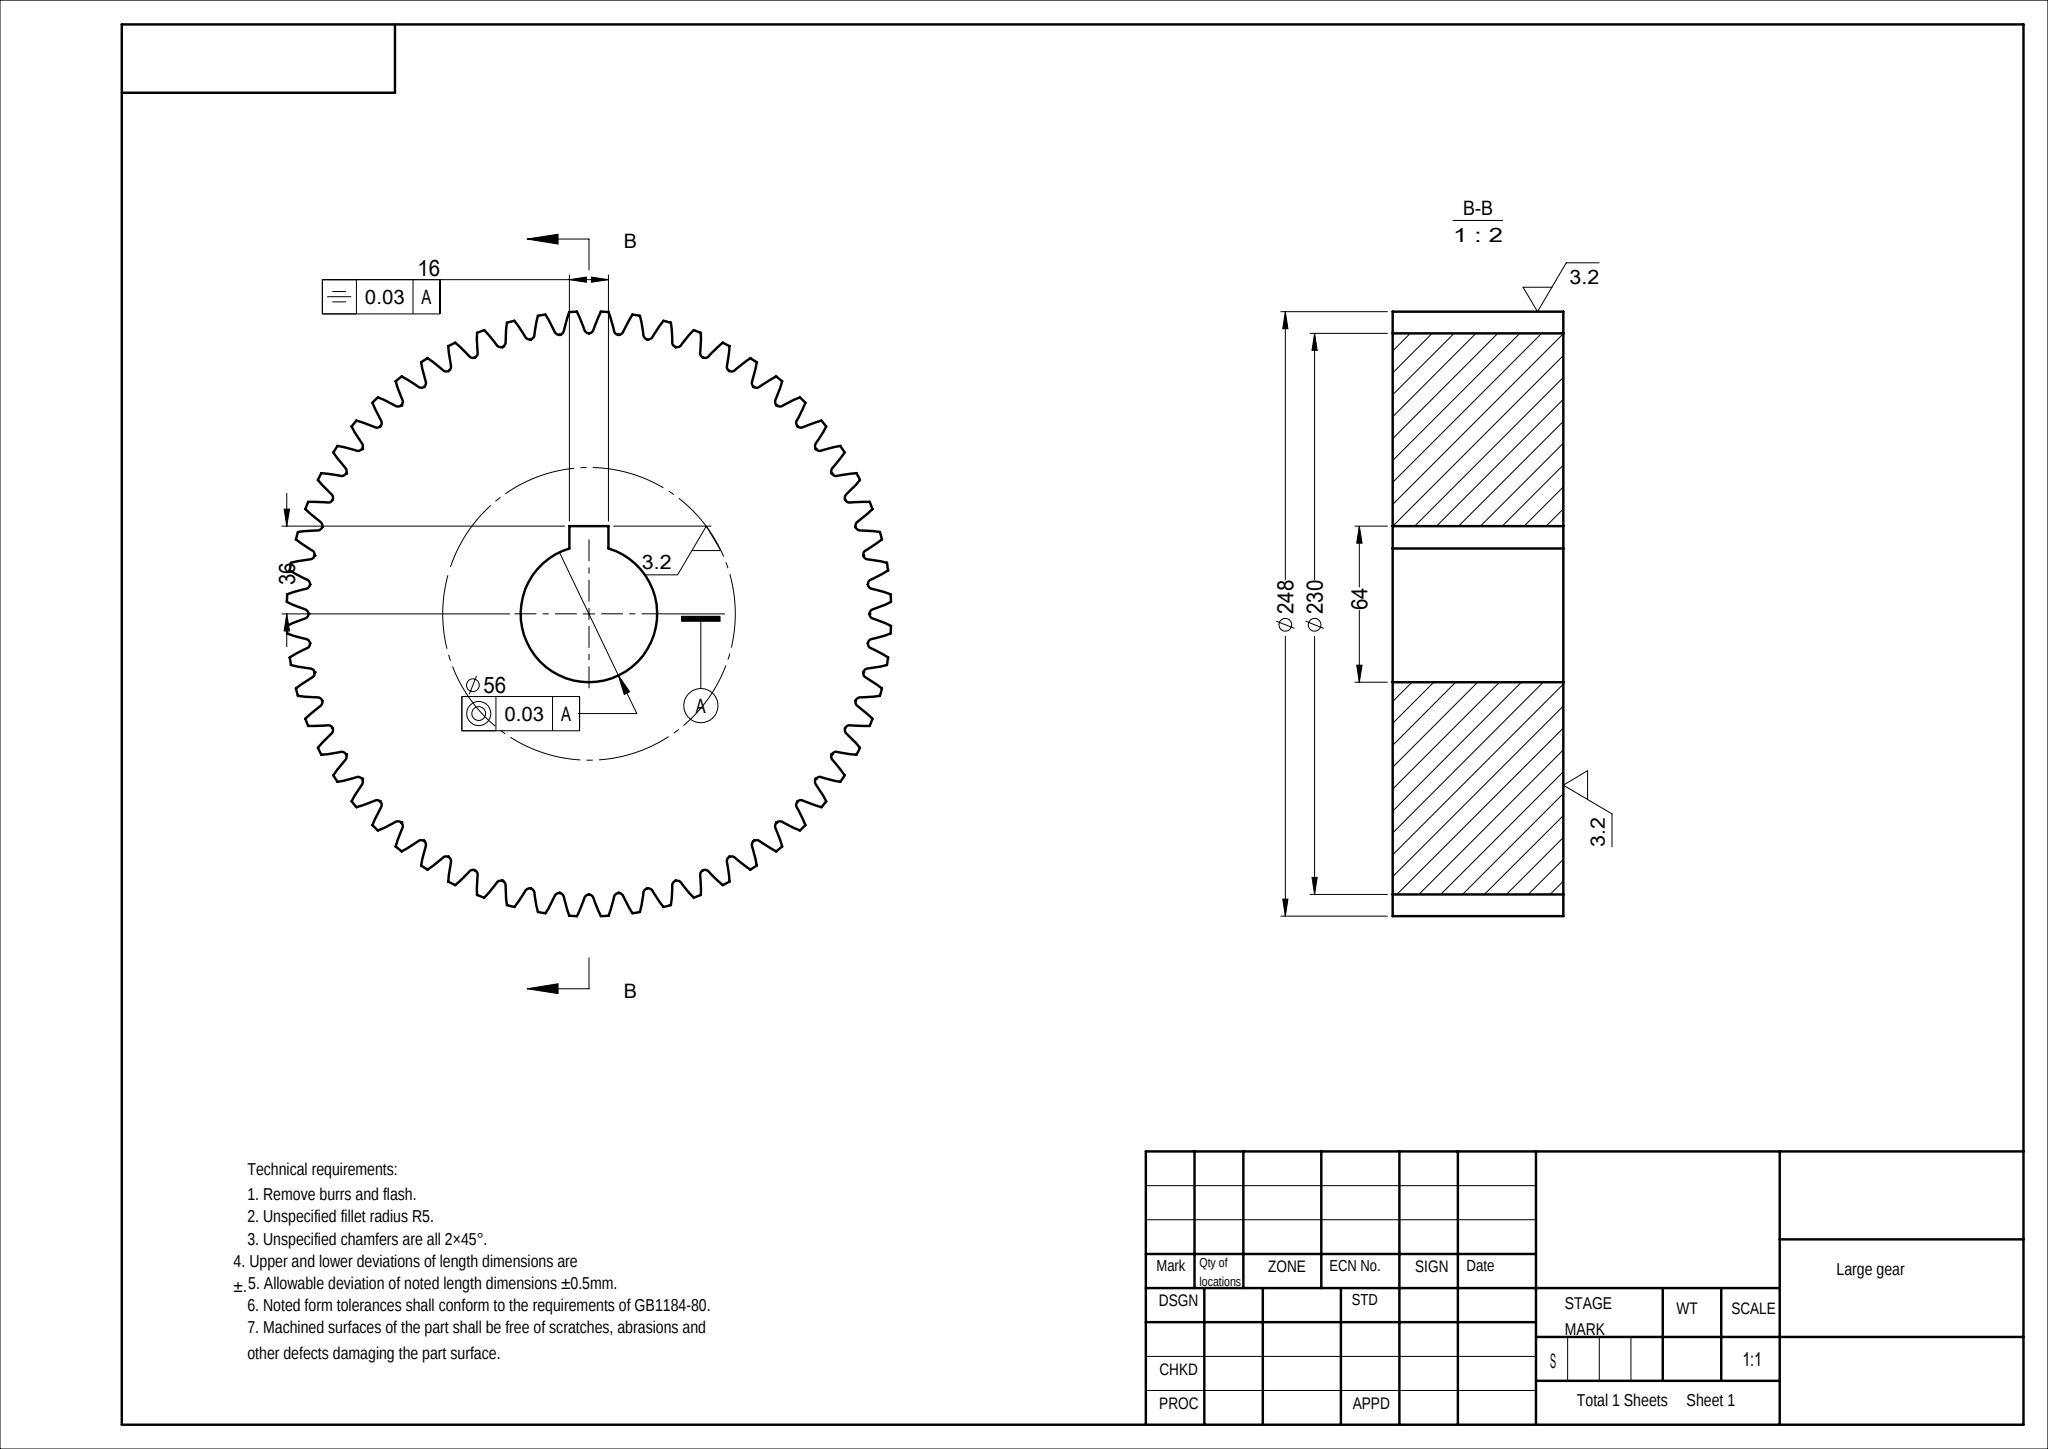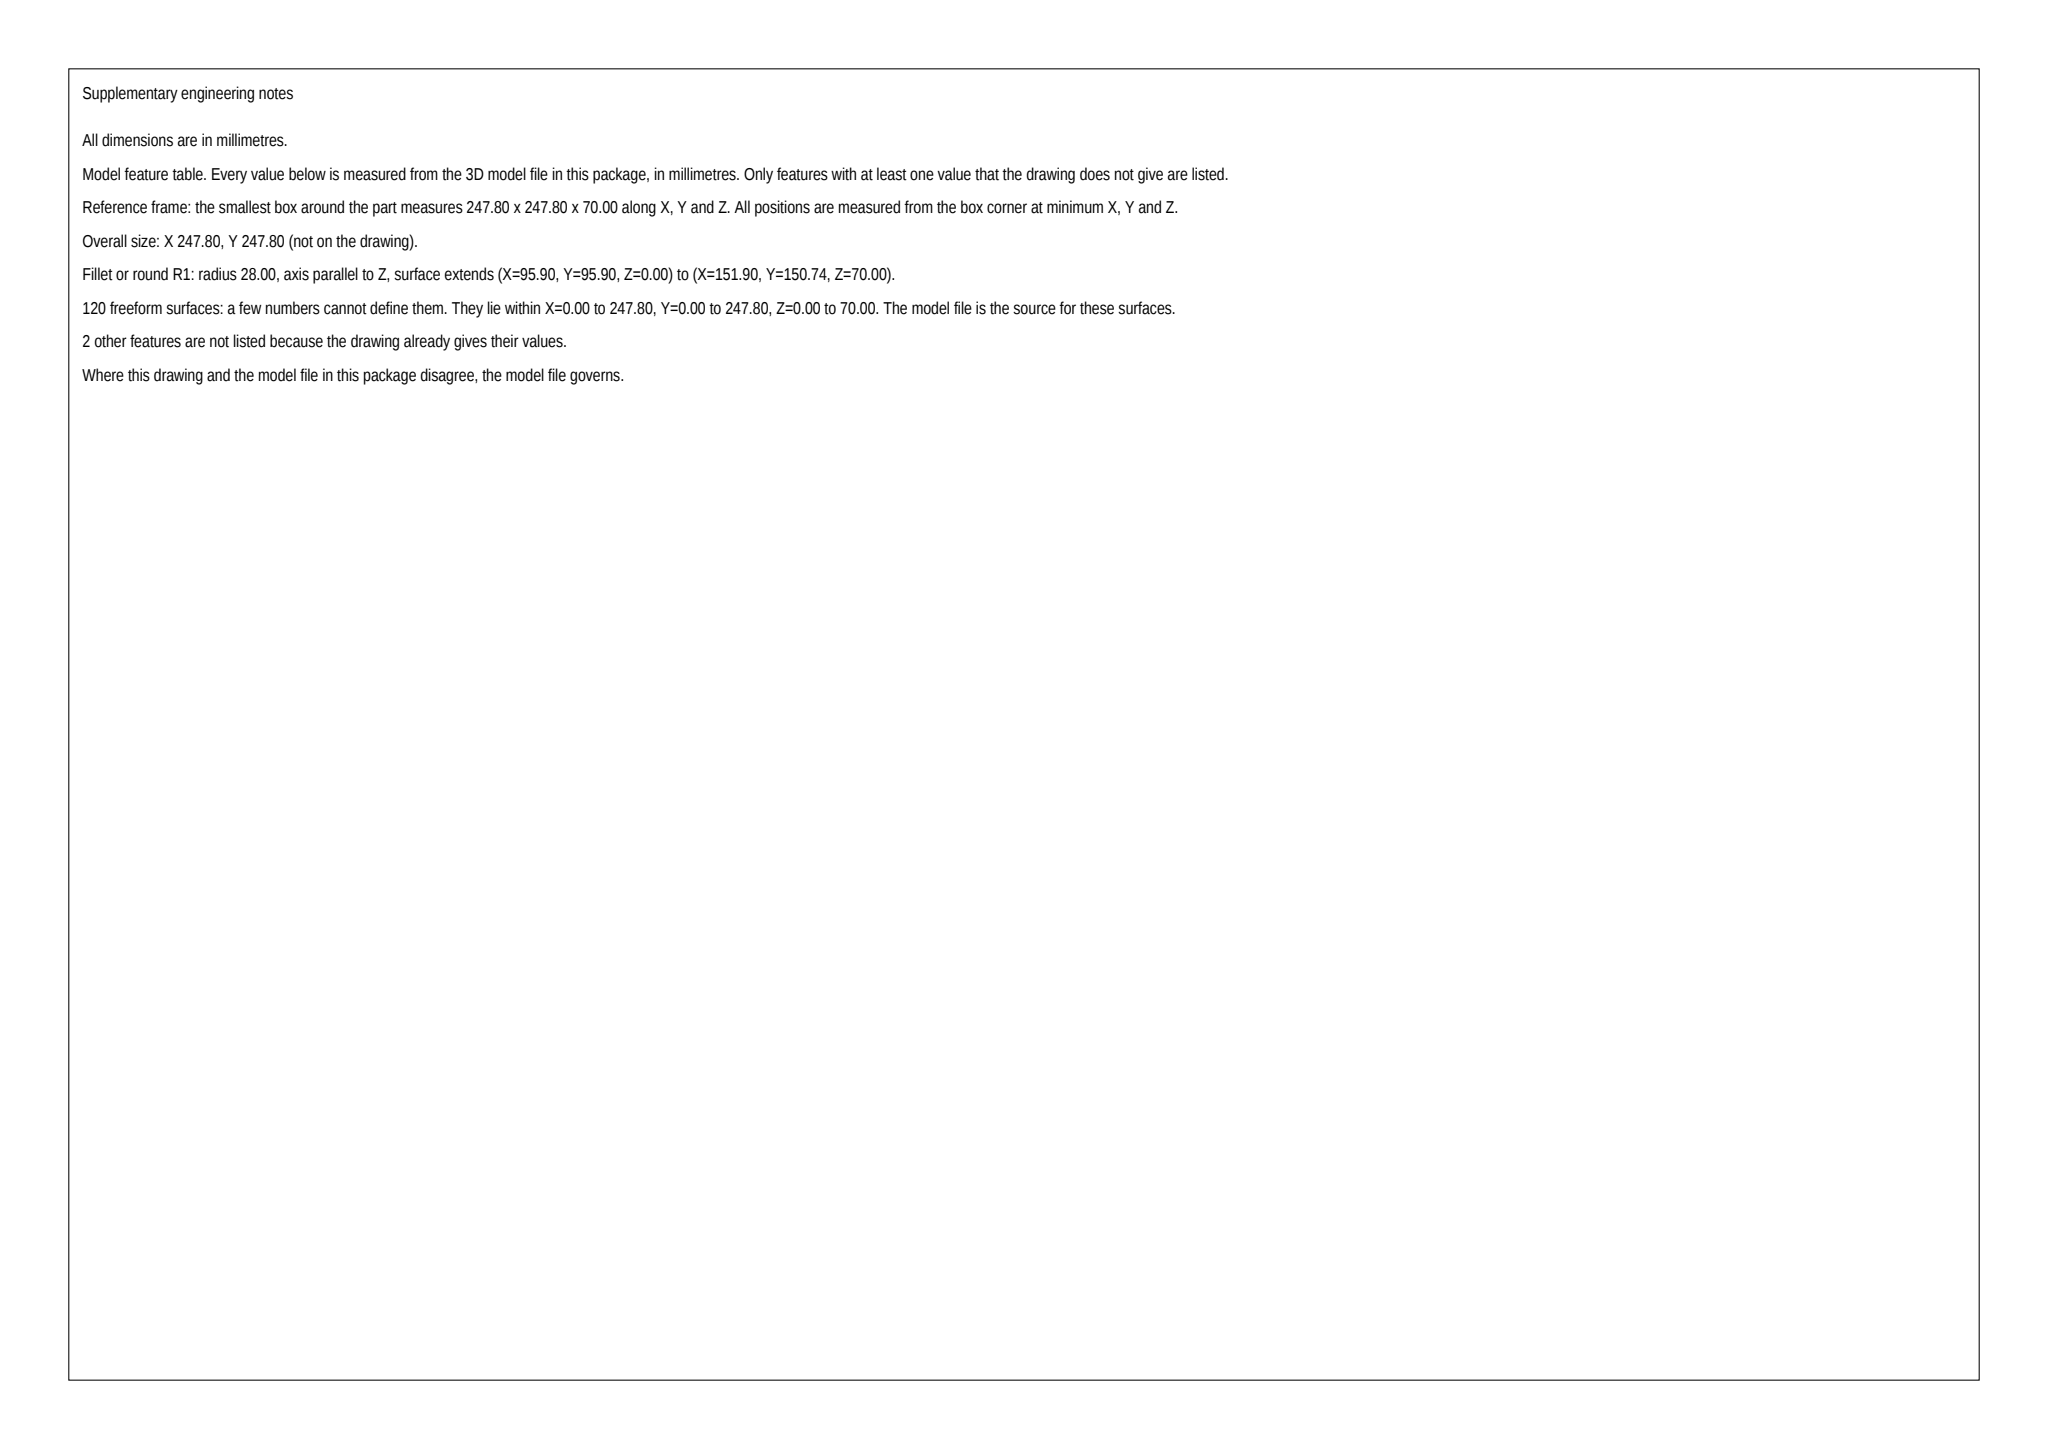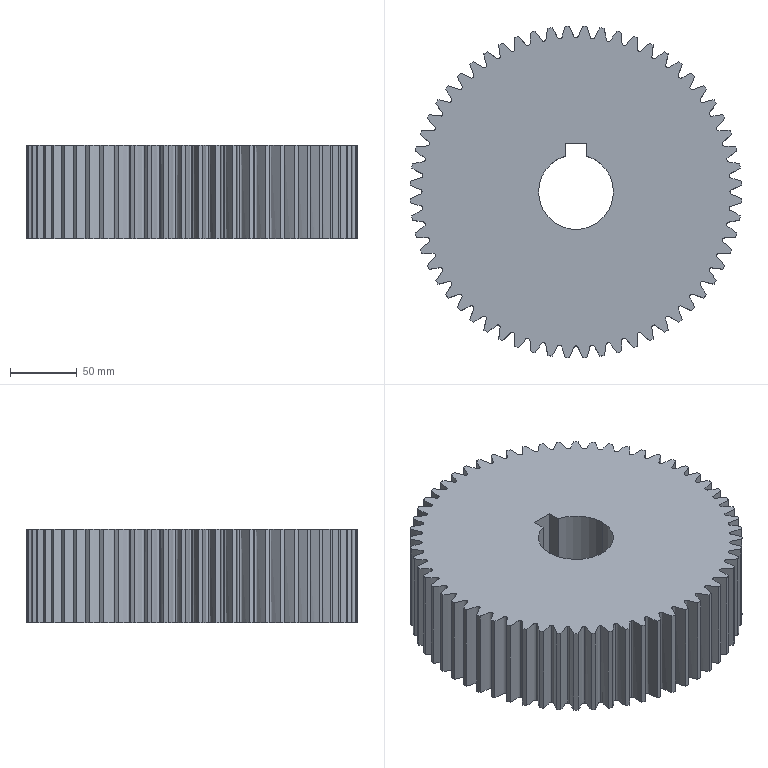Part | SolidWorks | mm | 1 solid | 248 faces | box 247.8 x 247.8 x 70 mm | volume 2975800 mm3 | cylinder 123 | spline 120 | plane 5 | commonest cylinder face diameters 248 x60 230 x60 56 x3